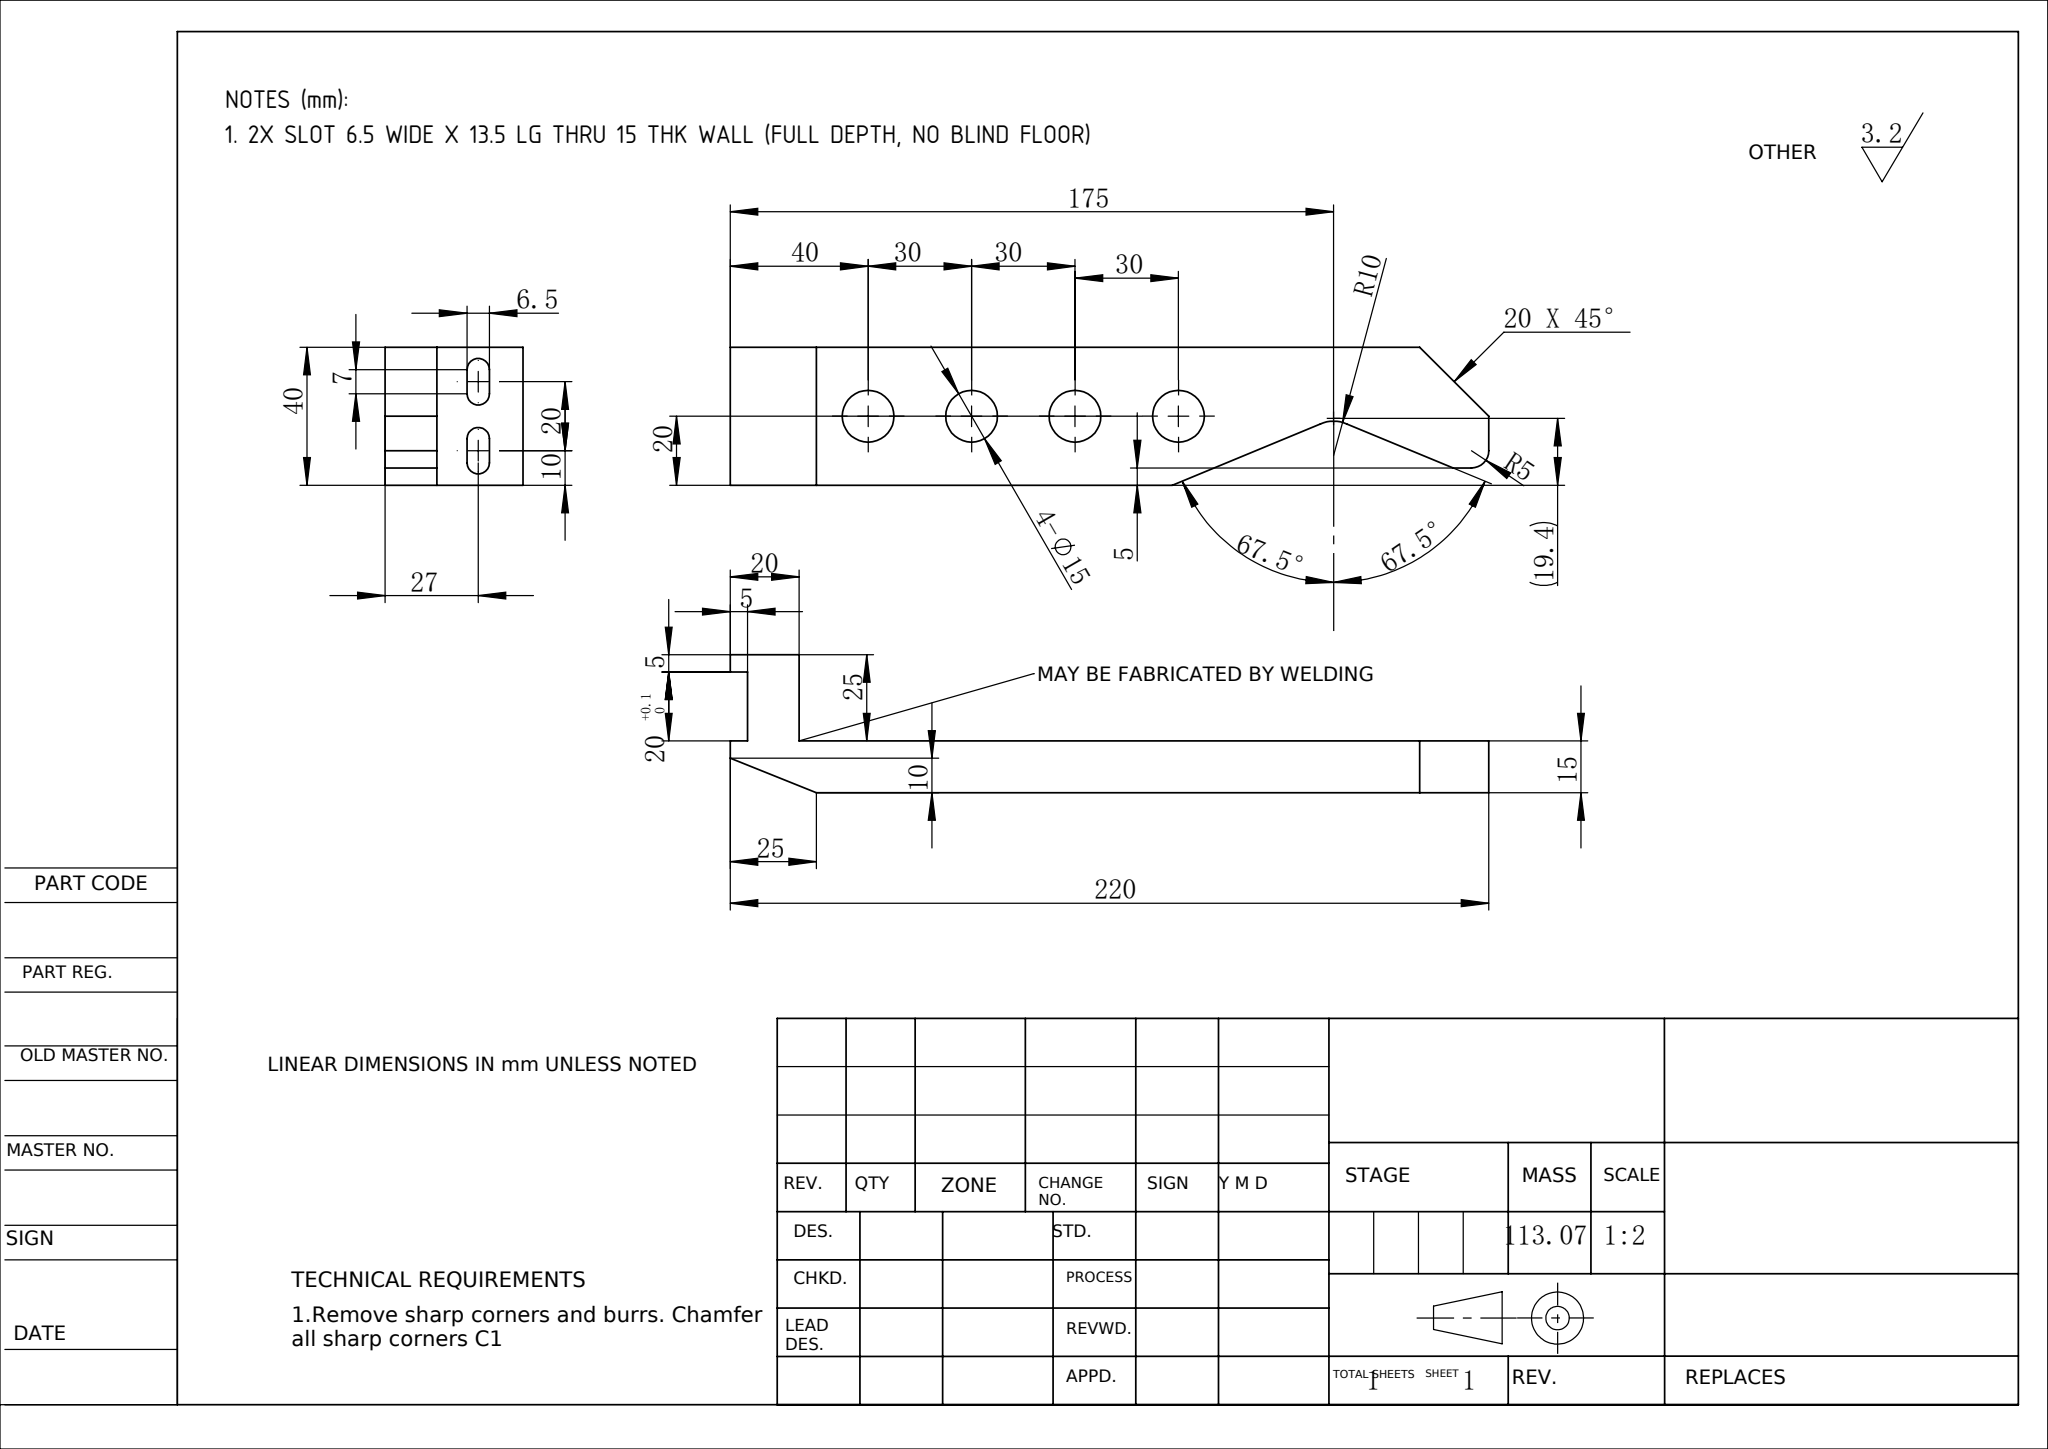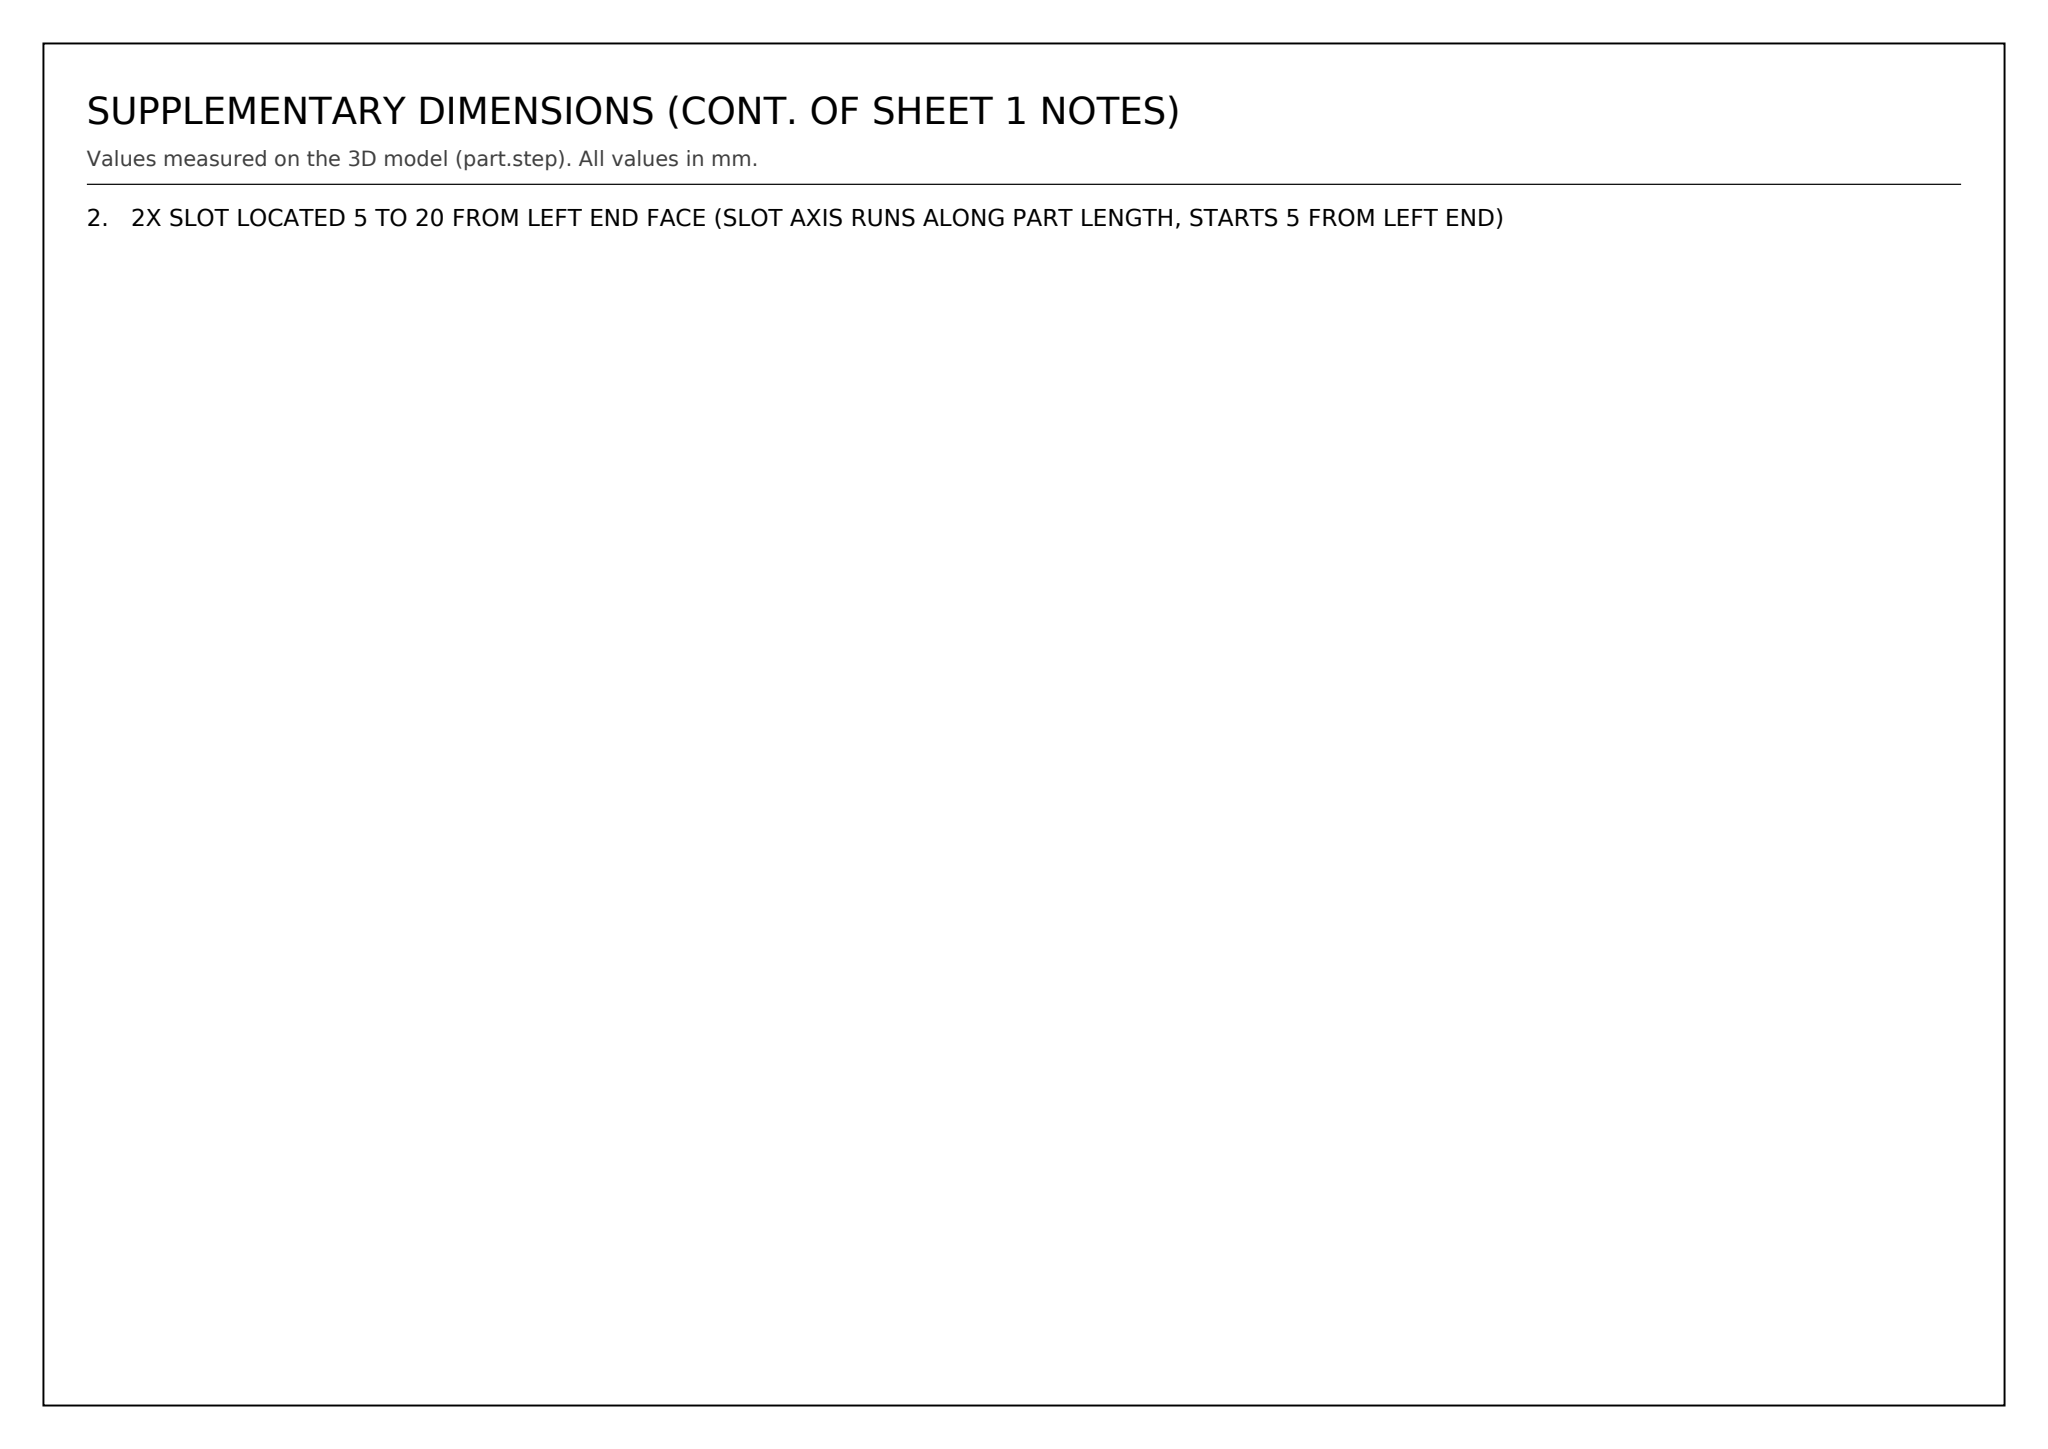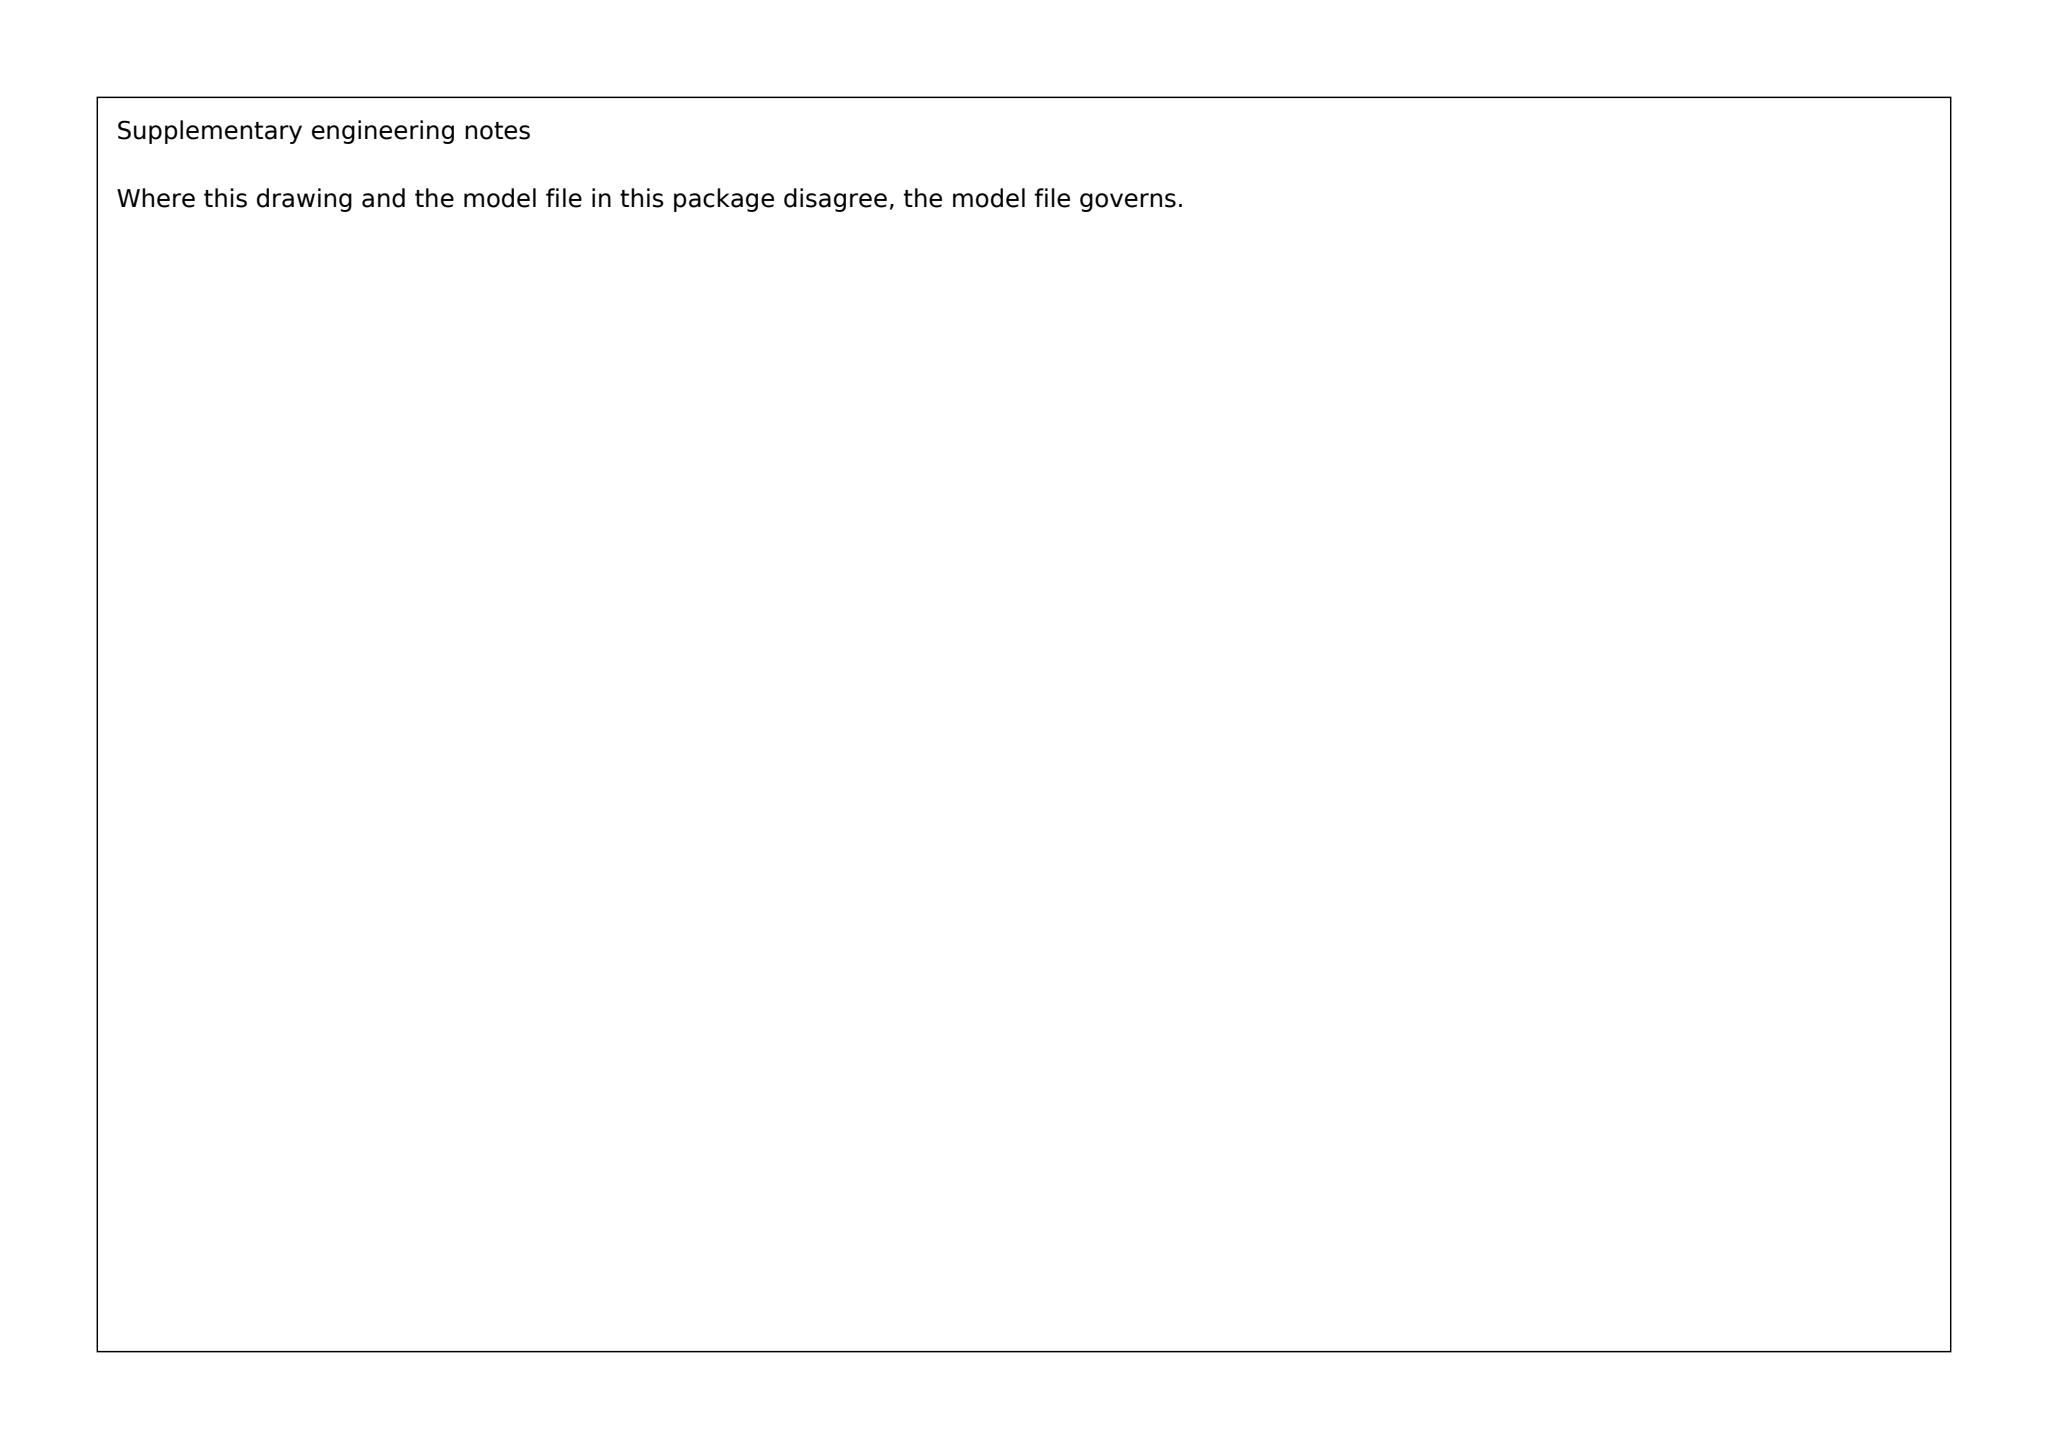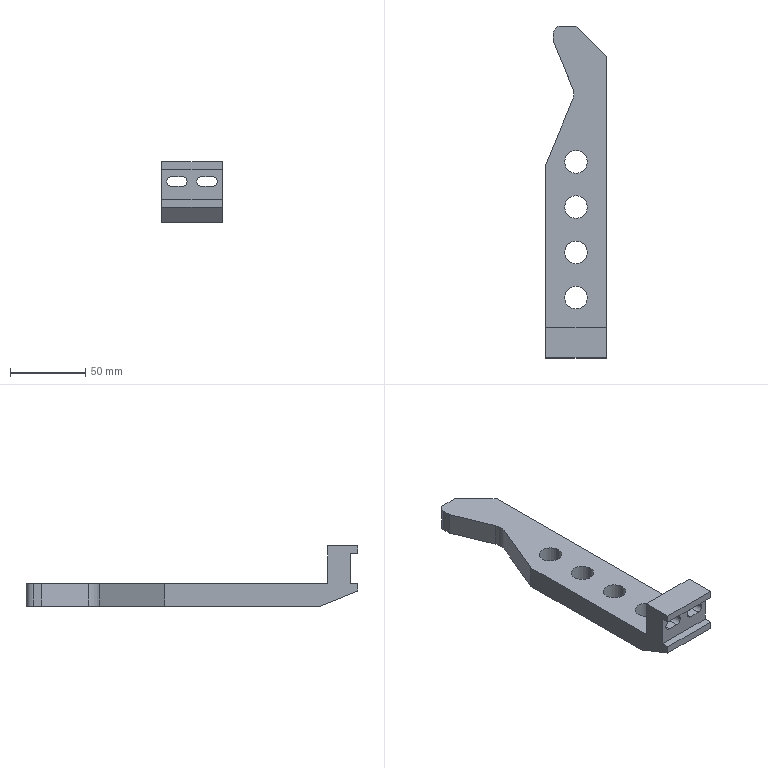Part | SolidWorks | mm | 1 solid | 37 faces | box 40 x 220 x 40 mm | volume 113071 mm3 | plane 21 | cylinder 16 | commonest cylinder face diameters 15 x8 6.5 x6 20 x1 10 x1
Drawing notes:
2X SLOT 6.5 WIDE X 13.5 LG THRU 15 THK WALL (FULL DEPTH, NO BLIND FLOOR) | from the solid: cylinders: 2 pairs of 6.5 dia concave arcs, axis y, from y=5.0 to y=20.0 (15 wall), end centres x=6.5/13.5 and x=26.5/33.5
2X SLOT LOCATED 5 TO 20 FROM LEFT END FACE (SLOT AXIS RUNS ALONG PART LENGTH, STARTS 5 FROM LEFT END) | from the solid: 6.5 dia slot-end cylinders axis y, from 5.0 to 20.0 measured from bbox min y (left end face); slot floor planes z=23.8/30.2 extent y [5.0, 20.0]
build123d program:
from build123d import *

# Parameters (mm, degrees)
BOSS_EXTRUDE1_DEPTH = 40
SKETCH2_W           = 25
SKETCH2_H           = 200
CUT_EXTRUDE1_DEPTH  = 223.317
SKETCH4_W           = 40
SKETCH4_H           = 40
BOSS_EXTRUDE2_DEPTH = 5
SKETCH5_W           = 40
SKETCH5_H           = 20
CUT_EXTRUDE3_DEPTH  = 5
CHAMFER1_SIZE       = 25
CHAMFER1_SIZE2      = 10
CUT_EXTRUDE6_DEPTH  = 223.317
CHAMFER2_SIZE       = 20
FILLET1_R           = 5
SKETCH12_R          = 7.5
CUT_EXTRUDE7_DEPTH  = 221.114


with BuildPart() as part:
    # Sketch1 → Boss-Extrude1 (new body)
    with BuildSketch(Plane.XY):
        with BuildLine():
            Line((40, 0), (0, 0))
            Line((0, 0), (0, 123.217))
            Line((0, 123.217), (17.793, 166.173))
            ThreePointArc((17.793, 166.173), (18.554, 170), (17.793, 173.827))
            Line((17.793, 173.827), (5, 204.712))
            Line((5, 204.712), (5, 215))
            Line((5, 215), (40, 215))
            Line((40, 215), (40, 0))
        make_face()
    extrude(amount=BOSS_EXTRUDE1_DEPTH)

    # Sketch2 → Cut-Extrude1 (cut, through all)
    with BuildSketch(Plane(origin=(40, 0, 0), x_dir=(0, 0, -1), z_dir=(1, 0, 0))):
        with Locations((-27.5, 115)):
            Rectangle(SKETCH2_W, SKETCH2_H)
    extrude(amount=-CUT_EXTRUDE1_DEPTH, mode=Mode.SUBTRACT)

    # Sketch4 → Boss-Extrude2 (add)
    with BuildSketch(Plane.XZ):
        with Locations((20, 20)):
            Rectangle(SKETCH4_W, SKETCH4_H)
    extrude(amount=BOSS_EXTRUDE2_DEPTH)

    # Sketch5 → Cut-Extrude3 (cut)
    with BuildSketch(Plane.XZ.offset(5)):
        with Locations((20, 25)):
            Rectangle(SKETCH5_W, SKETCH5_H)
    extrude(amount=-CUT_EXTRUDE3_DEPTH, mode=Mode.SUBTRACT)

    # Chamfer1
    chamfer1_edges = [part.edges().sort_by_distance(p)[0] for p in [
        (20, -5, 0),
    ]]
    chamfer1_side = [part.faces().sort_by_distance(p)[0] for p in [
        (21.603, 97.247, 0),
    ]]
    chamfer(chamfer1_edges, length=CHAMFER1_SIZE, length2=CHAMFER1_SIZE2, reference=chamfer1_side[0])

    # Sketch9 → Cut-Extrude6 (cut, through all)
    with BuildSketch(Plane.XZ):
        with BuildLine():
            Line((13.5, 23.75), (6.5, 23.75))
            ThreePointArc((6.5, 23.75), (3.25, 27), (6.5, 30.25))
            Line((6.5, 30.25), (13.5, 30.25))
            ThreePointArc((13.5, 30.25), (16.75, 27), (13.5, 23.75))
        make_face()
        with BuildLine():
            Line((33.5, 23.75), (26.5, 23.75))
            ThreePointArc((26.5, 23.75), (23.25, 27), (26.5, 30.25))
            Line((26.5, 30.25), (33.5, 30.25))
            ThreePointArc((33.5, 30.25), (36.75, 27), (33.5, 23.75))
        make_face()
    extrude(amount=-CUT_EXTRUDE6_DEPTH, mode=Mode.SUBTRACT)

    # Chamfer2
    chamfer2_edges = [part.edges().sort_by_distance(p)[0] for p in [
        (40, 215, 7.5),
    ]]
    chamfer(chamfer2_edges, length=CHAMFER2_SIZE)

    # Fillet1
    fillet1_edges = [part.edges().sort_by_distance(p)[0] for p in [
        (5, 215, 7.5),
    ]]
    fillet(fillet1_edges, radius=FILLET1_R)

    # Sketch12 → Cut-Extrude7 (cut, through all)
    with BuildSketch(Plane.XY.offset(15)):
        with Locations((20, 35)):
            Circle(SKETCH12_R)
        with Locations((20, 65)):
            Circle(SKETCH12_R)
        with Locations((20, 95)):
            Circle(SKETCH12_R)
        with Locations((20, 125)):
            Circle(SKETCH12_R)
    extrude(amount=-CUT_EXTRUDE7_DEPTH, mode=Mode.SUBTRACT)


solid = part.part